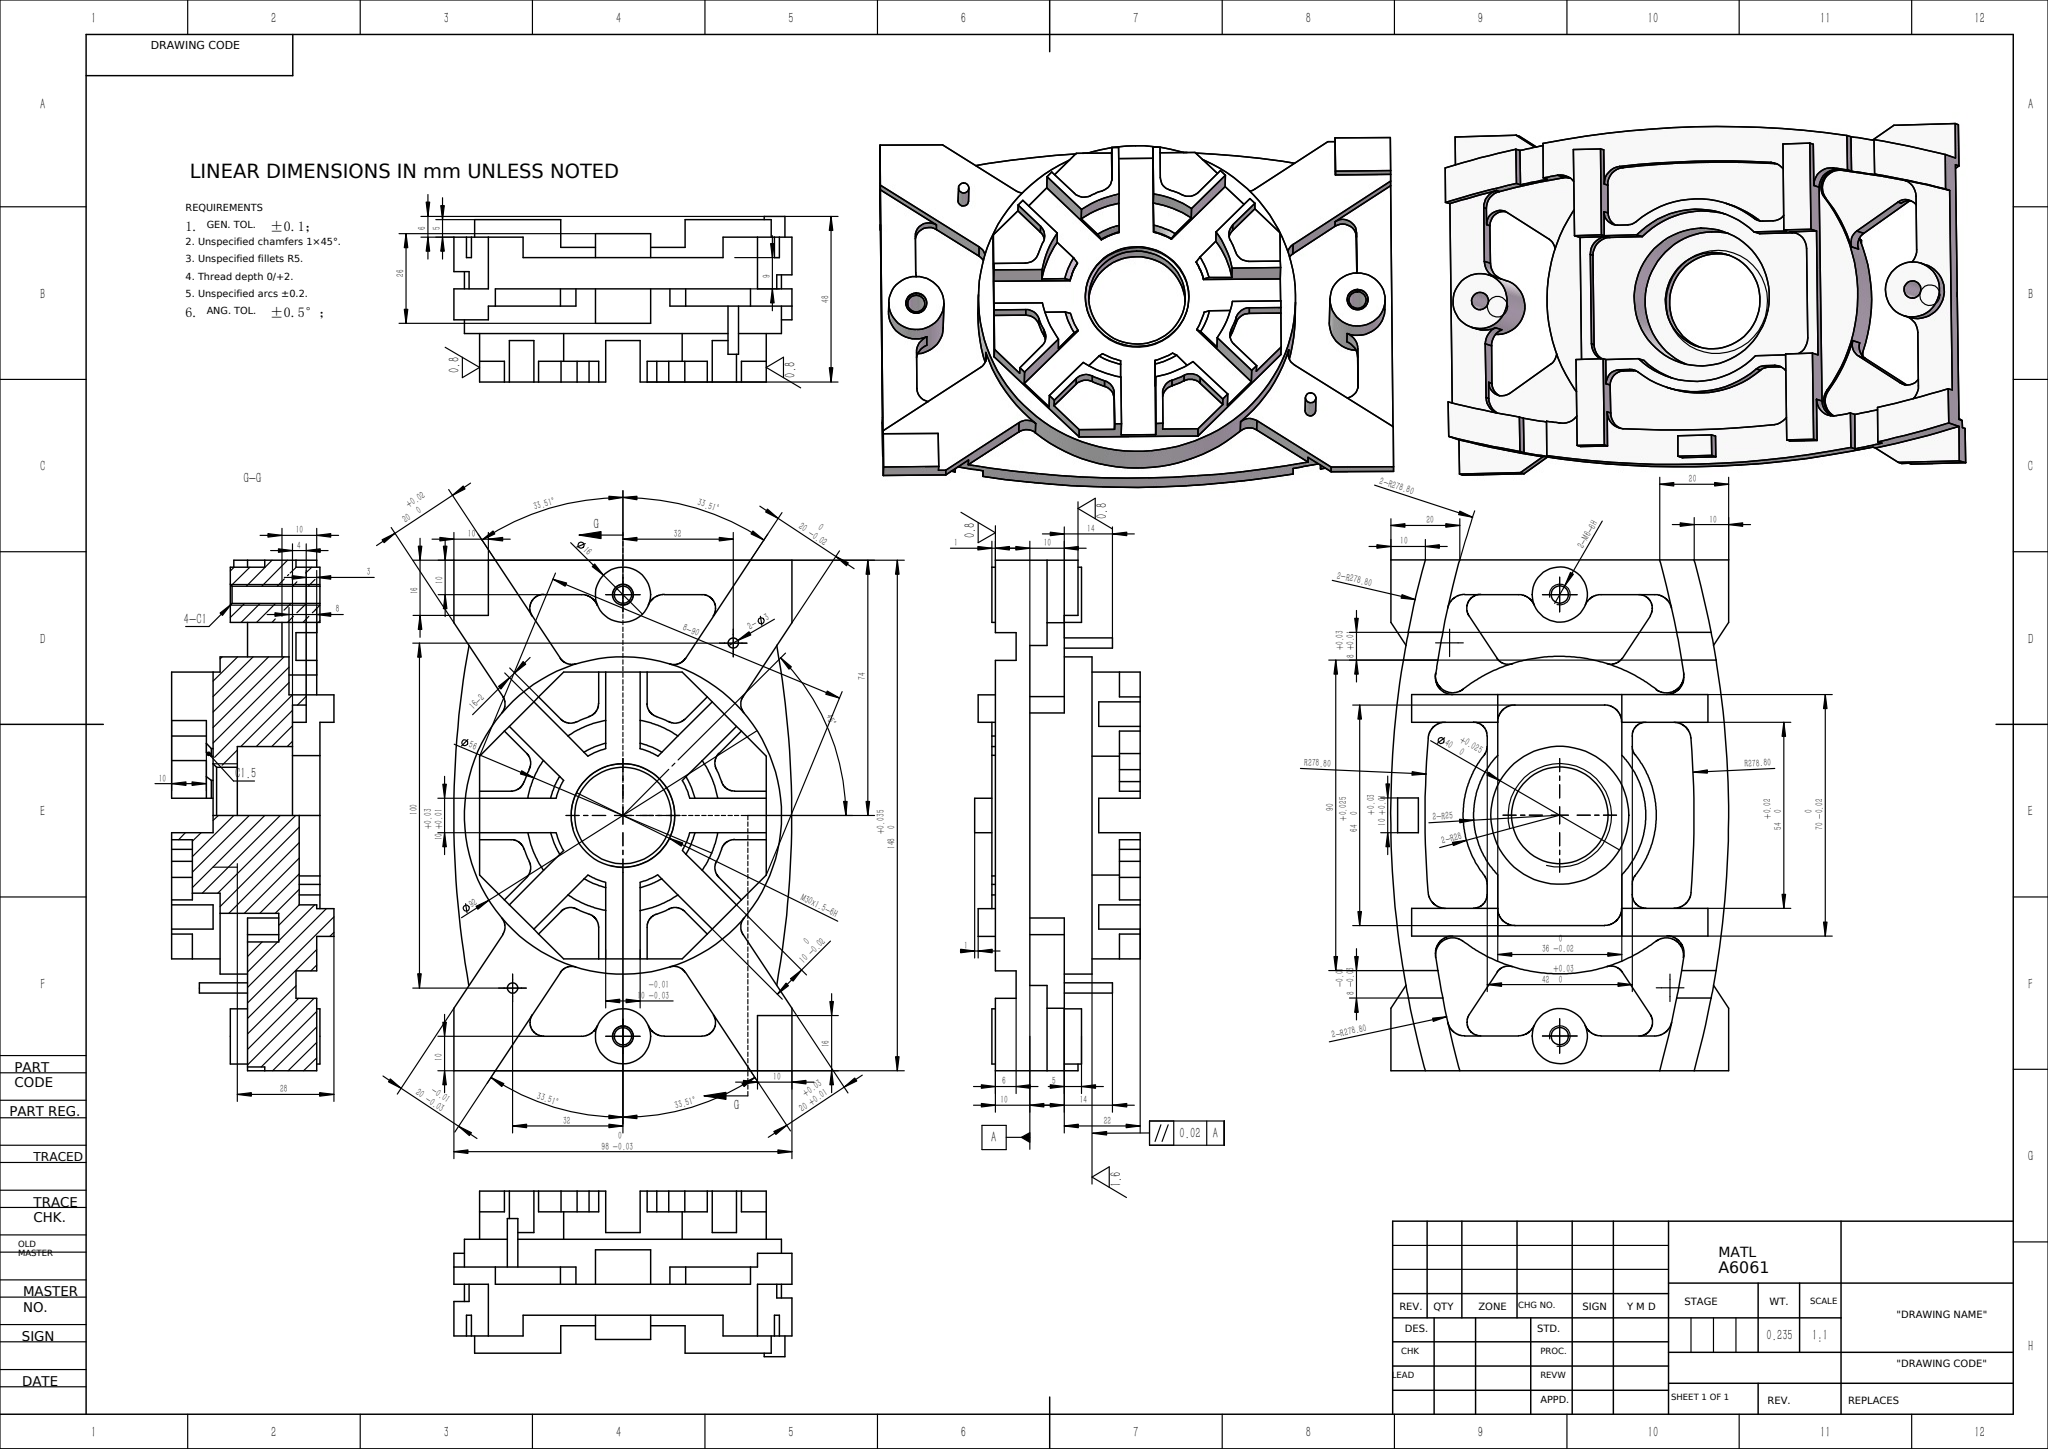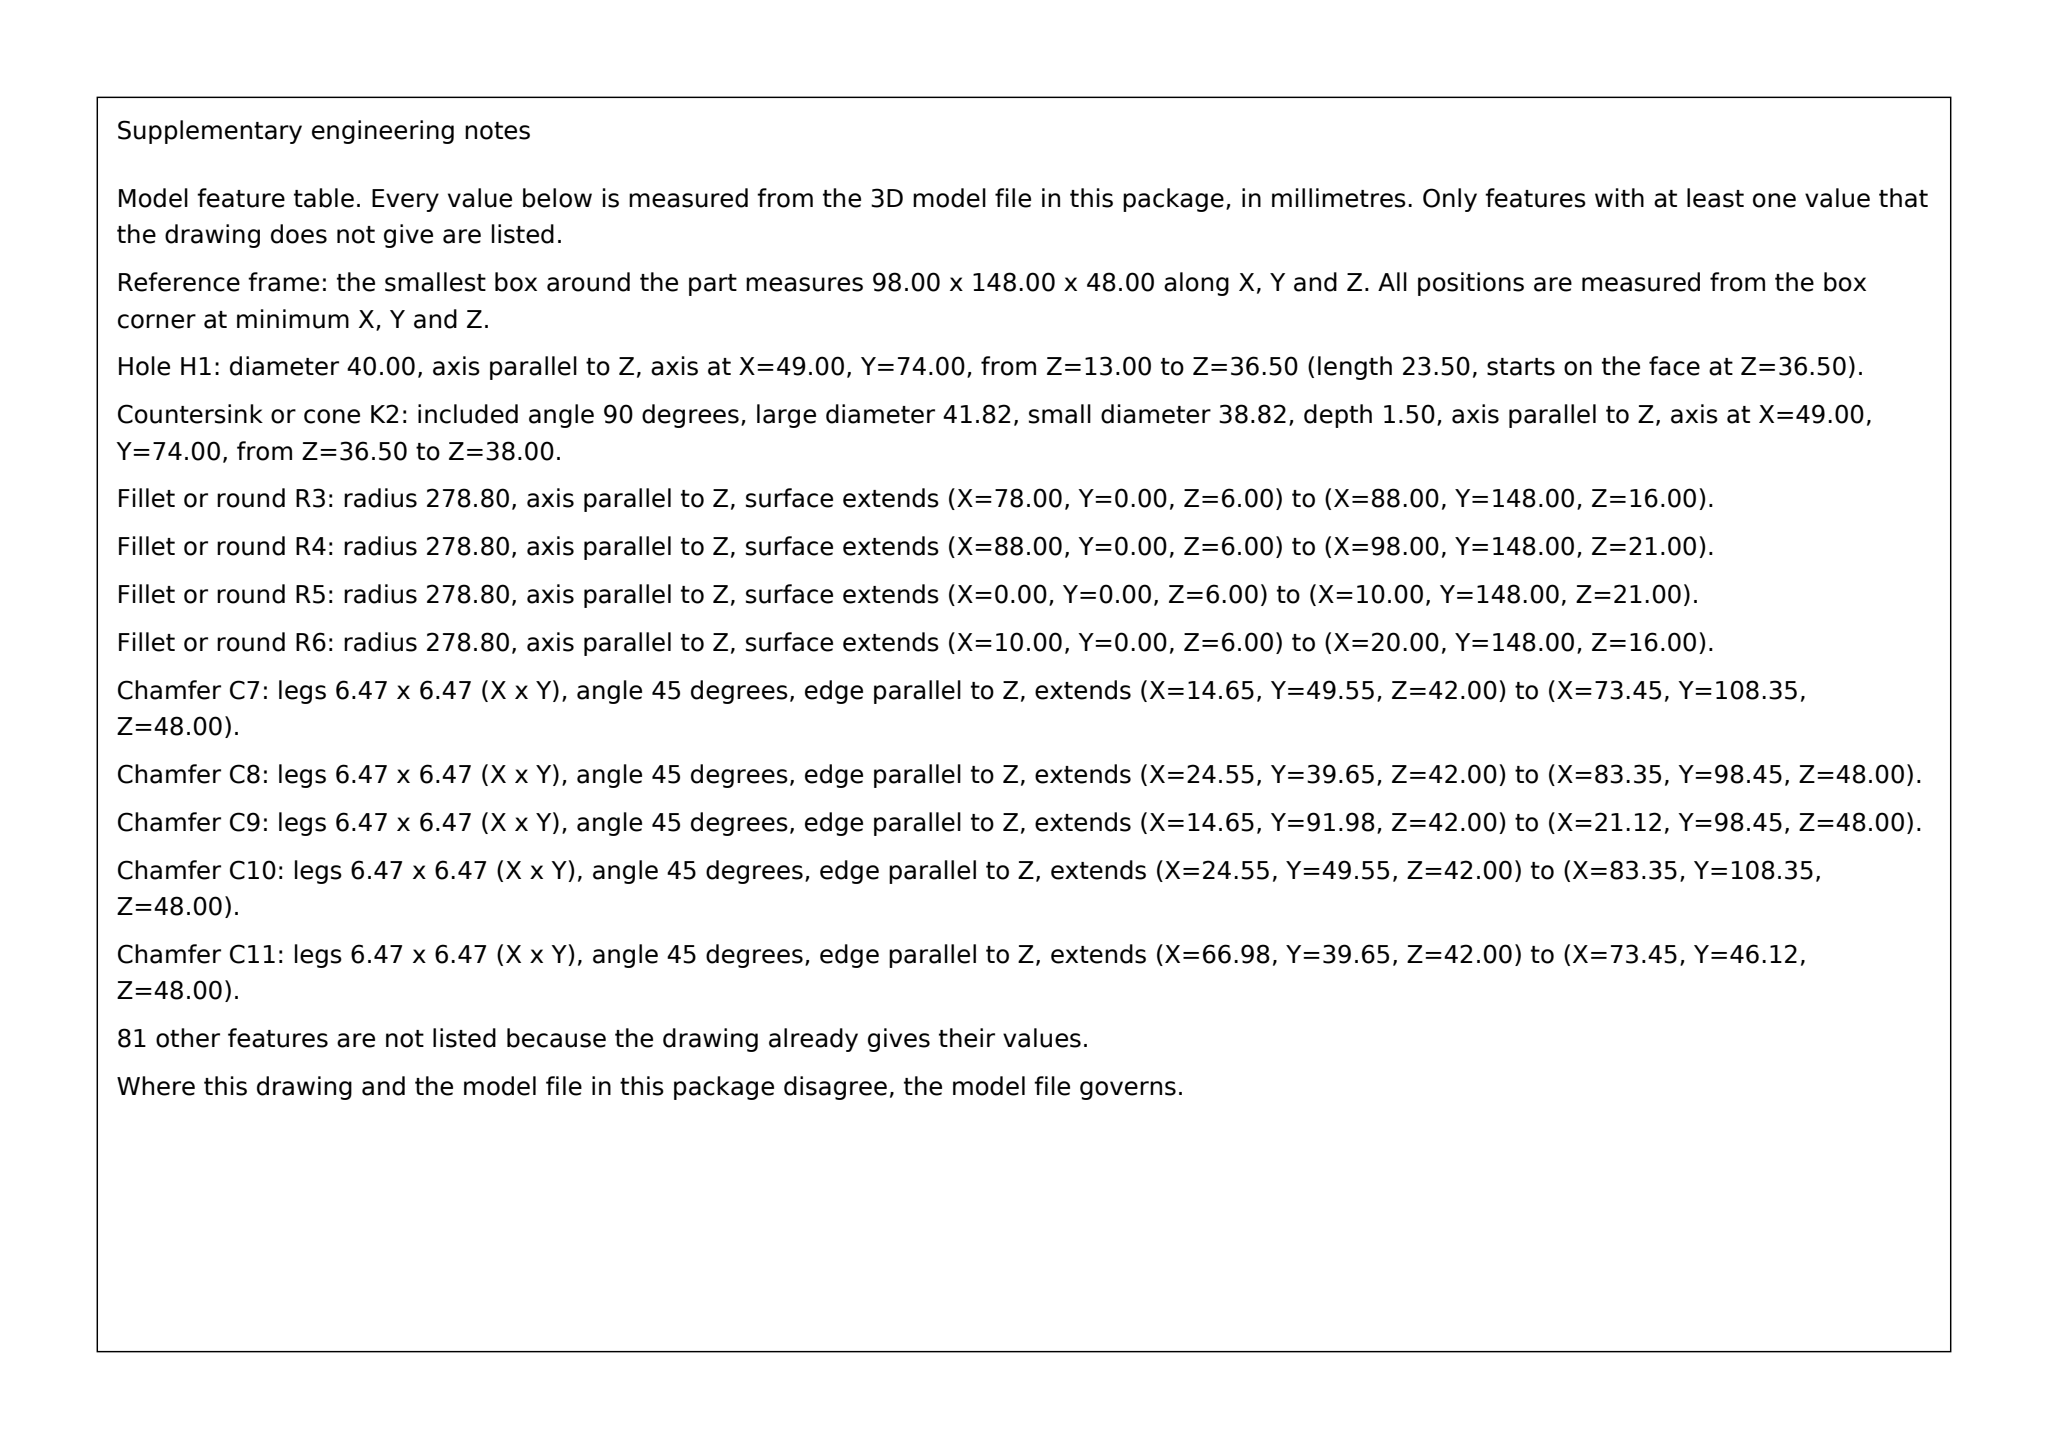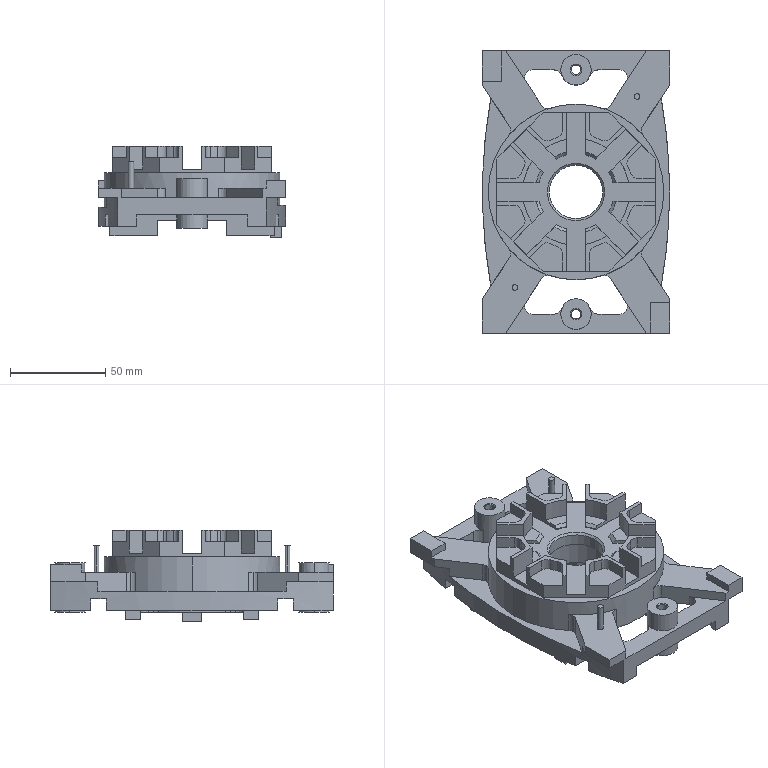Part | SolidWorks | mm | material A6061 | 1 solid | 315 faces | box 98 x 148 x 48 mm | volume 234929 mm3 | plane 171 | cylinder 130 | cone 14 | commonest cylinder face diameters 8 x42 10 x28 56 x11 40 x10 557.6 x10 44 x8 16 x6 5 x4